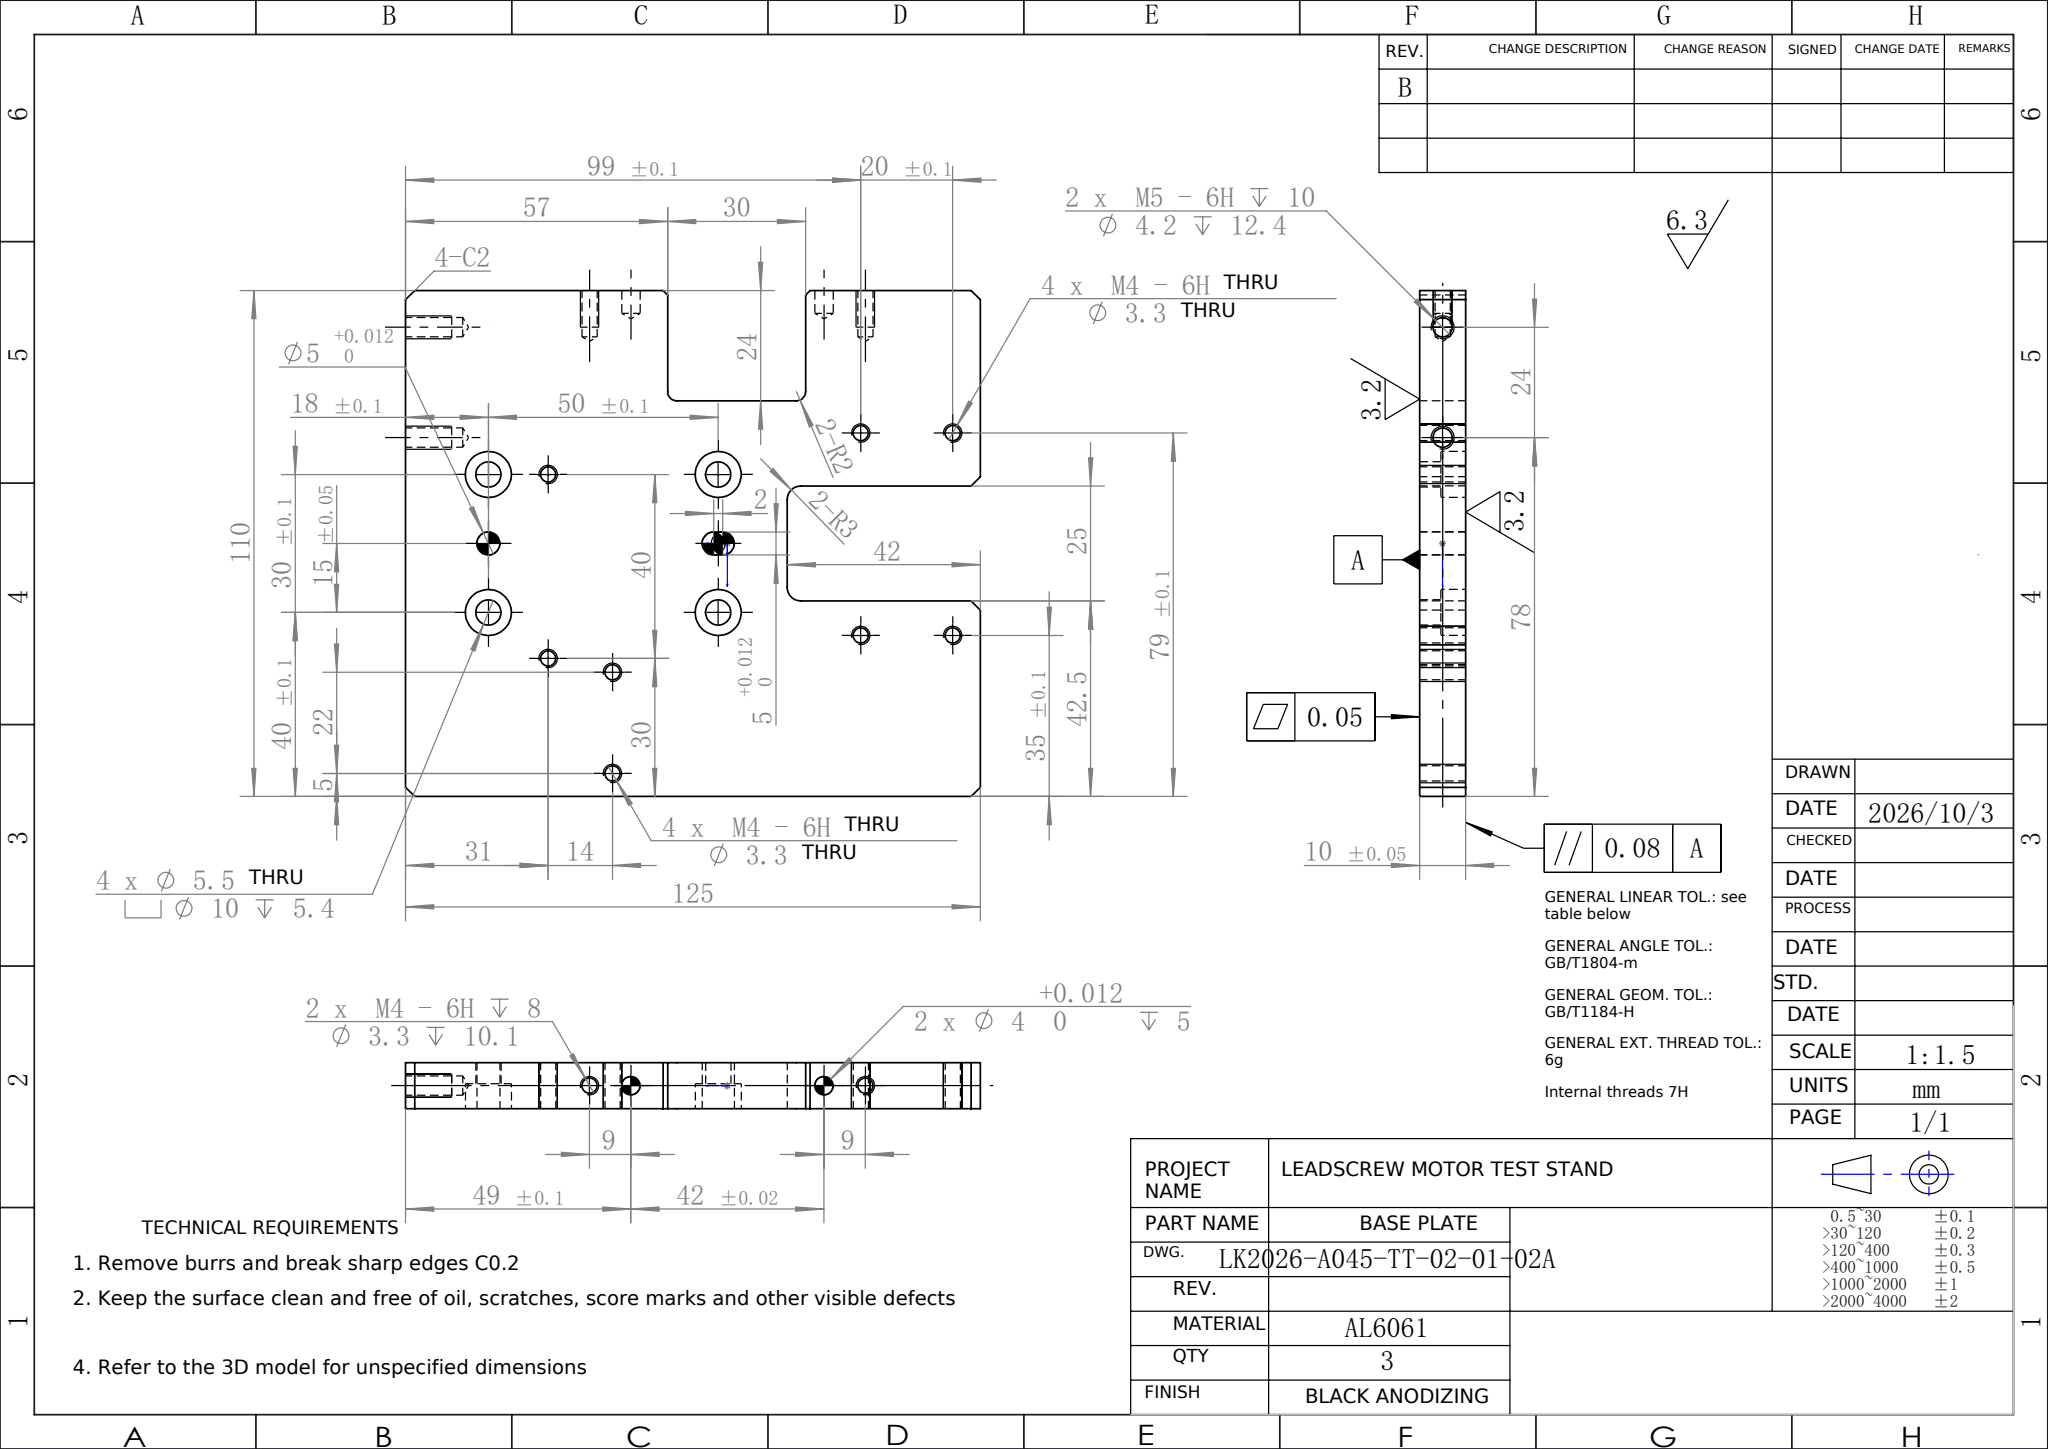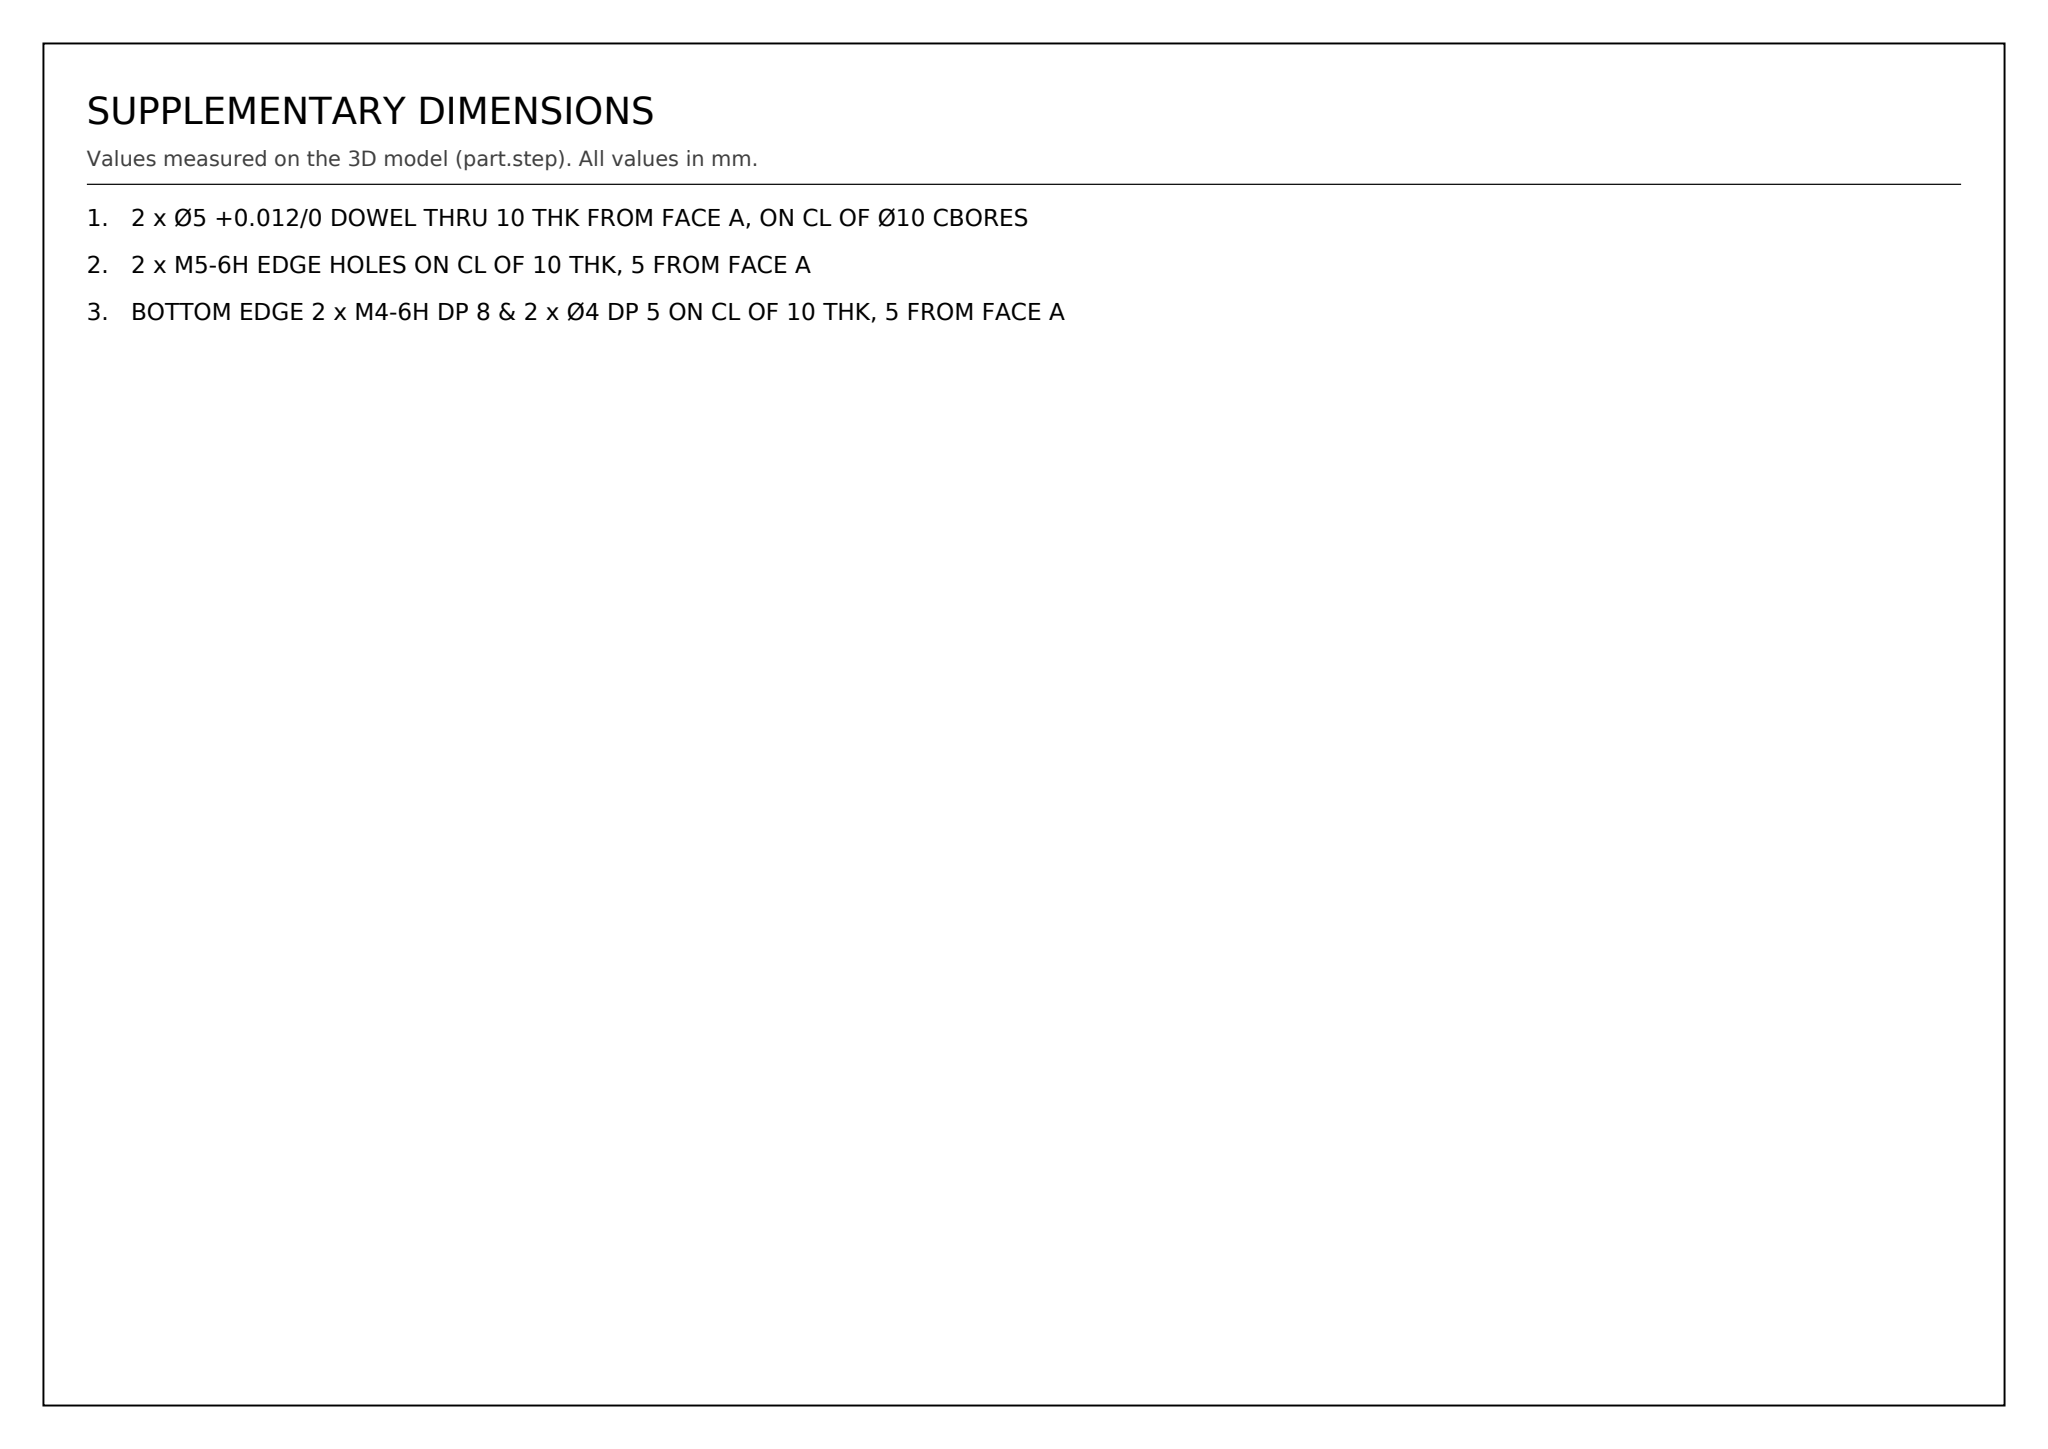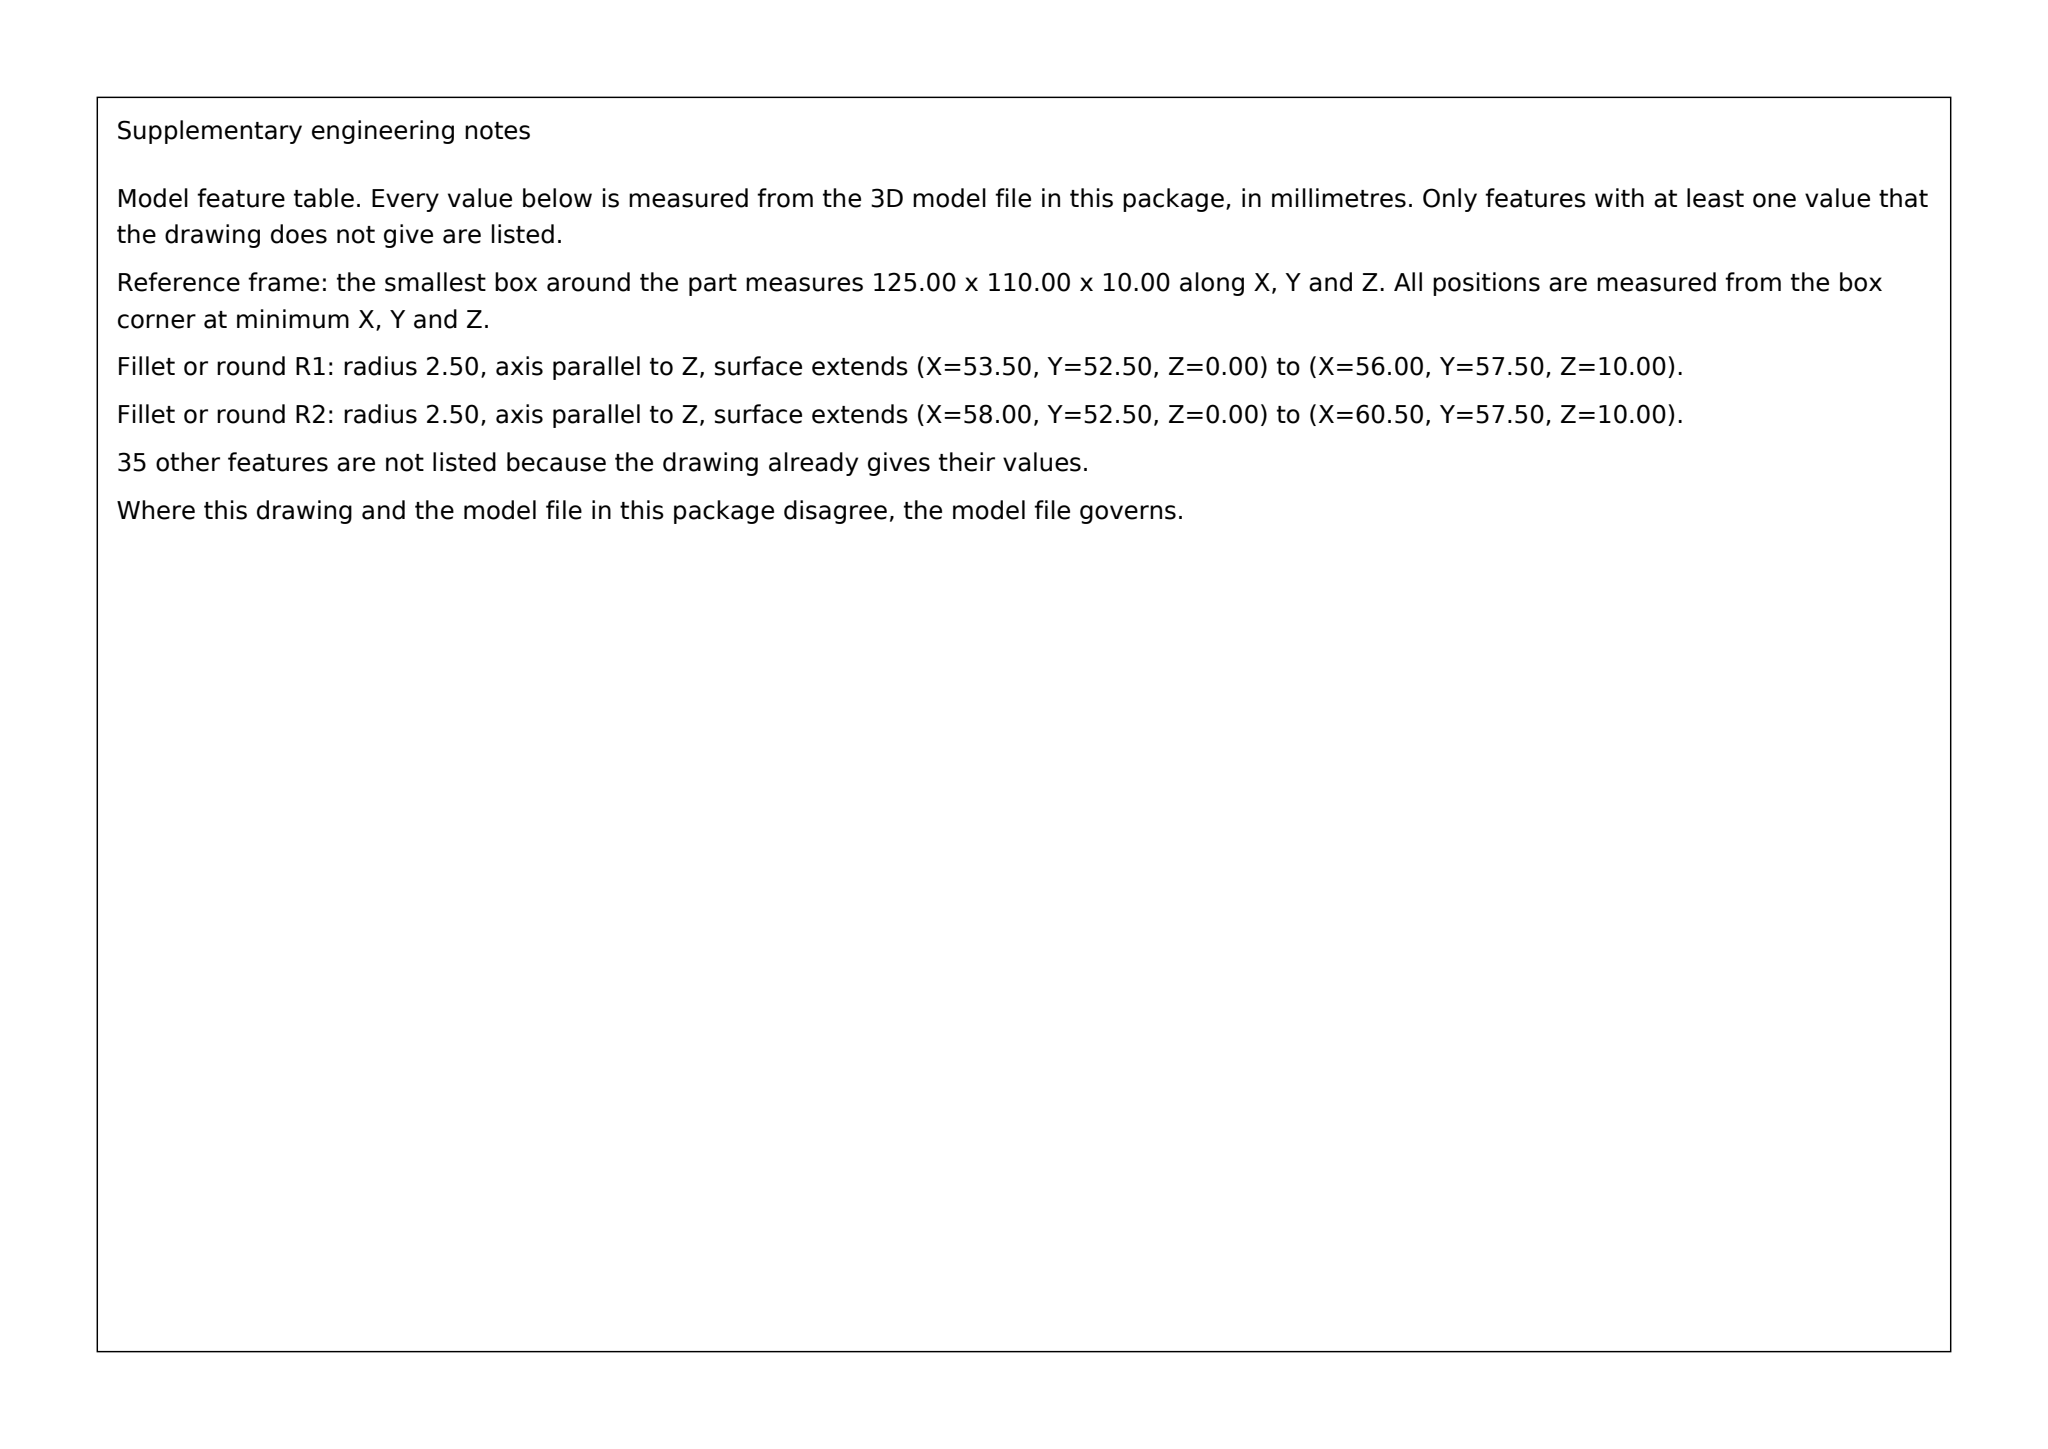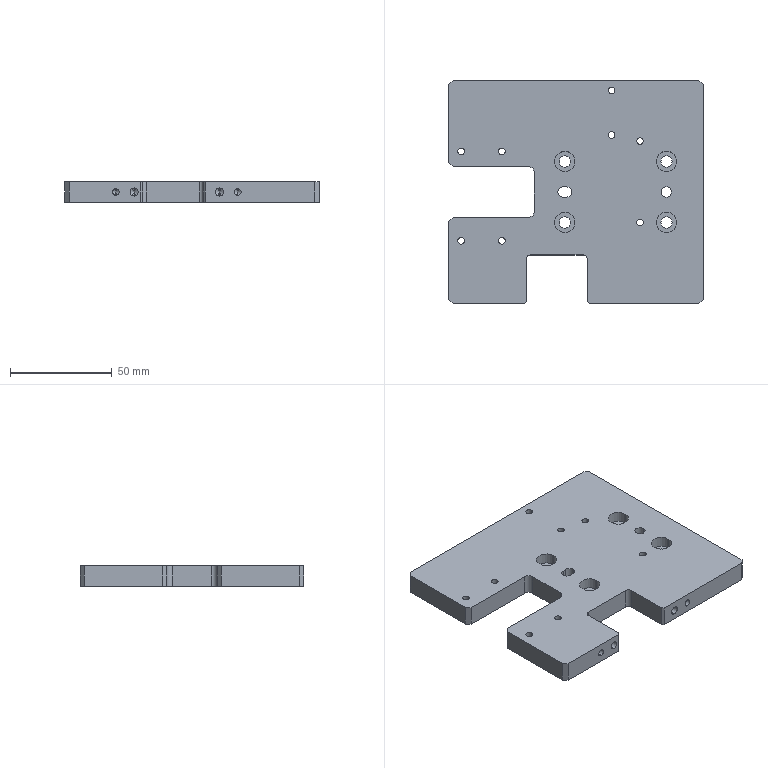Part | SolidWorks | mm | 1 solid | 93 faces | box 125 x 110 x 10 mm | volume 115746 mm3 | cylinder 53 | plane 28 | cone 12 | commonest cylinder face diameters 3.3 x20 10 x8 5.5 x8 4 x6 5 x5 4.2 x4 6 x2
Drawing notes:
2 x Ø5 +0.012/0 DOWEL THRU 10 THK FROM FACE A, ON CL OF Ø10 CBORES | from the solid: Ø5 z-axis cyls L=10.0 = full plate thk; at x=107 & x=57, y=55, coaxial with Ø10 cbores
2 x M5-6H EDGE HOLES ON CL OF 10 THK, 5 FROM FACE A | from the solid: Ø4.2 x-axis cyls at [-,8.0,5.0] & [-,32.0,5.0], L=12.4; plate z=0-10 so axis z=5 = mid-thk
BOTTOM EDGE 2 x M4-6H DP 8 & 2 x Ø4 DP 5 ON CL OF 10 THK, 5 FROM FACE A | from the solid: Ø3.3 y-axis cyls at [25,-,5] & [85,-,5] L=10.1; Ø4 y-axis cyls at [34,-,5] & [76,-,5] L=5